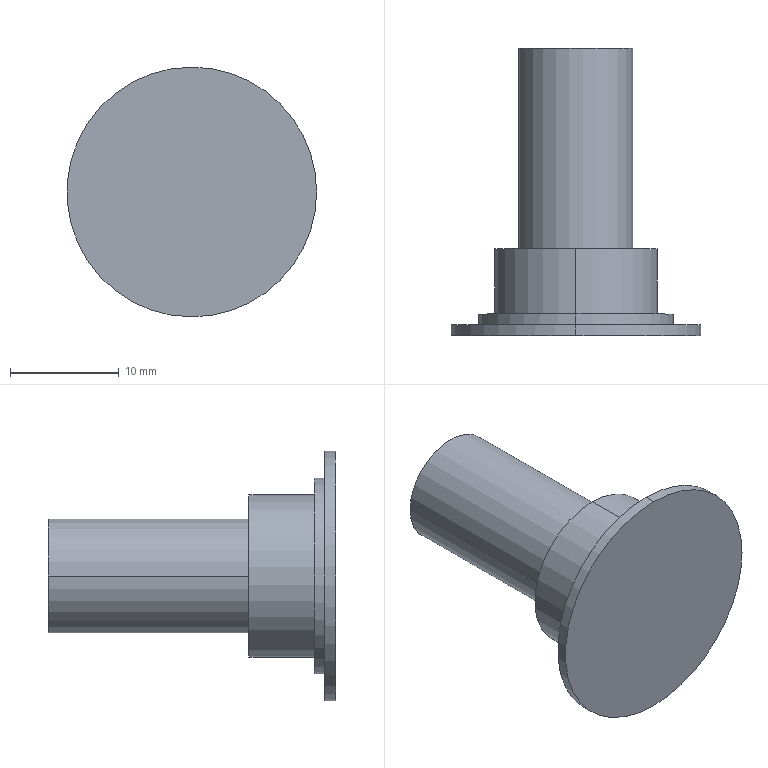CAM job | Mastercam | mm | 3 operations | part box 23 x 26.5 x 23
1. Drill/Counterbore | 7 - 4 倒角刀
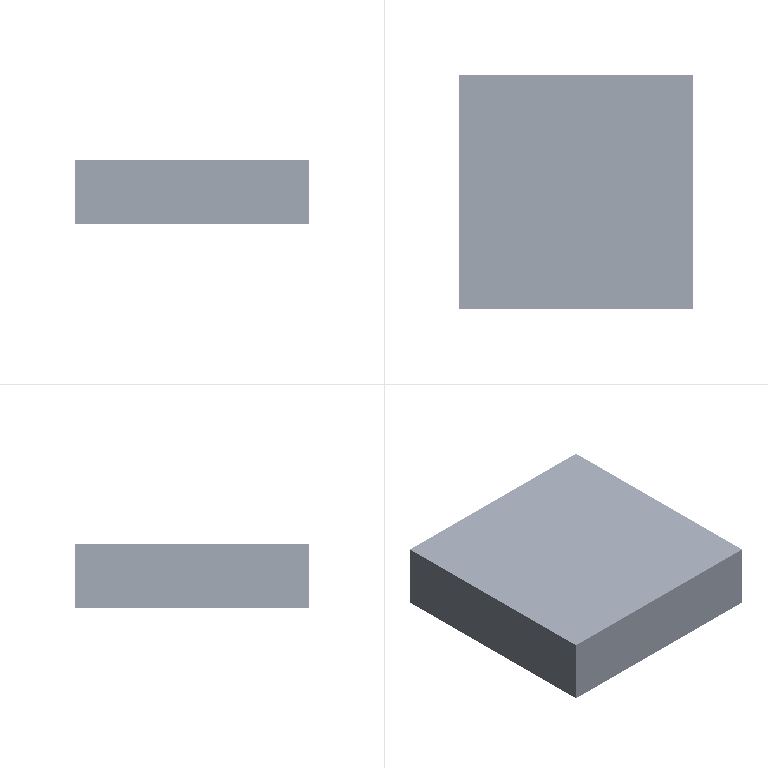2. Contour (Ramp) | 10 - 10 平铣刀
3. Contour (2D chamfer) | 7 - 4 倒角刀